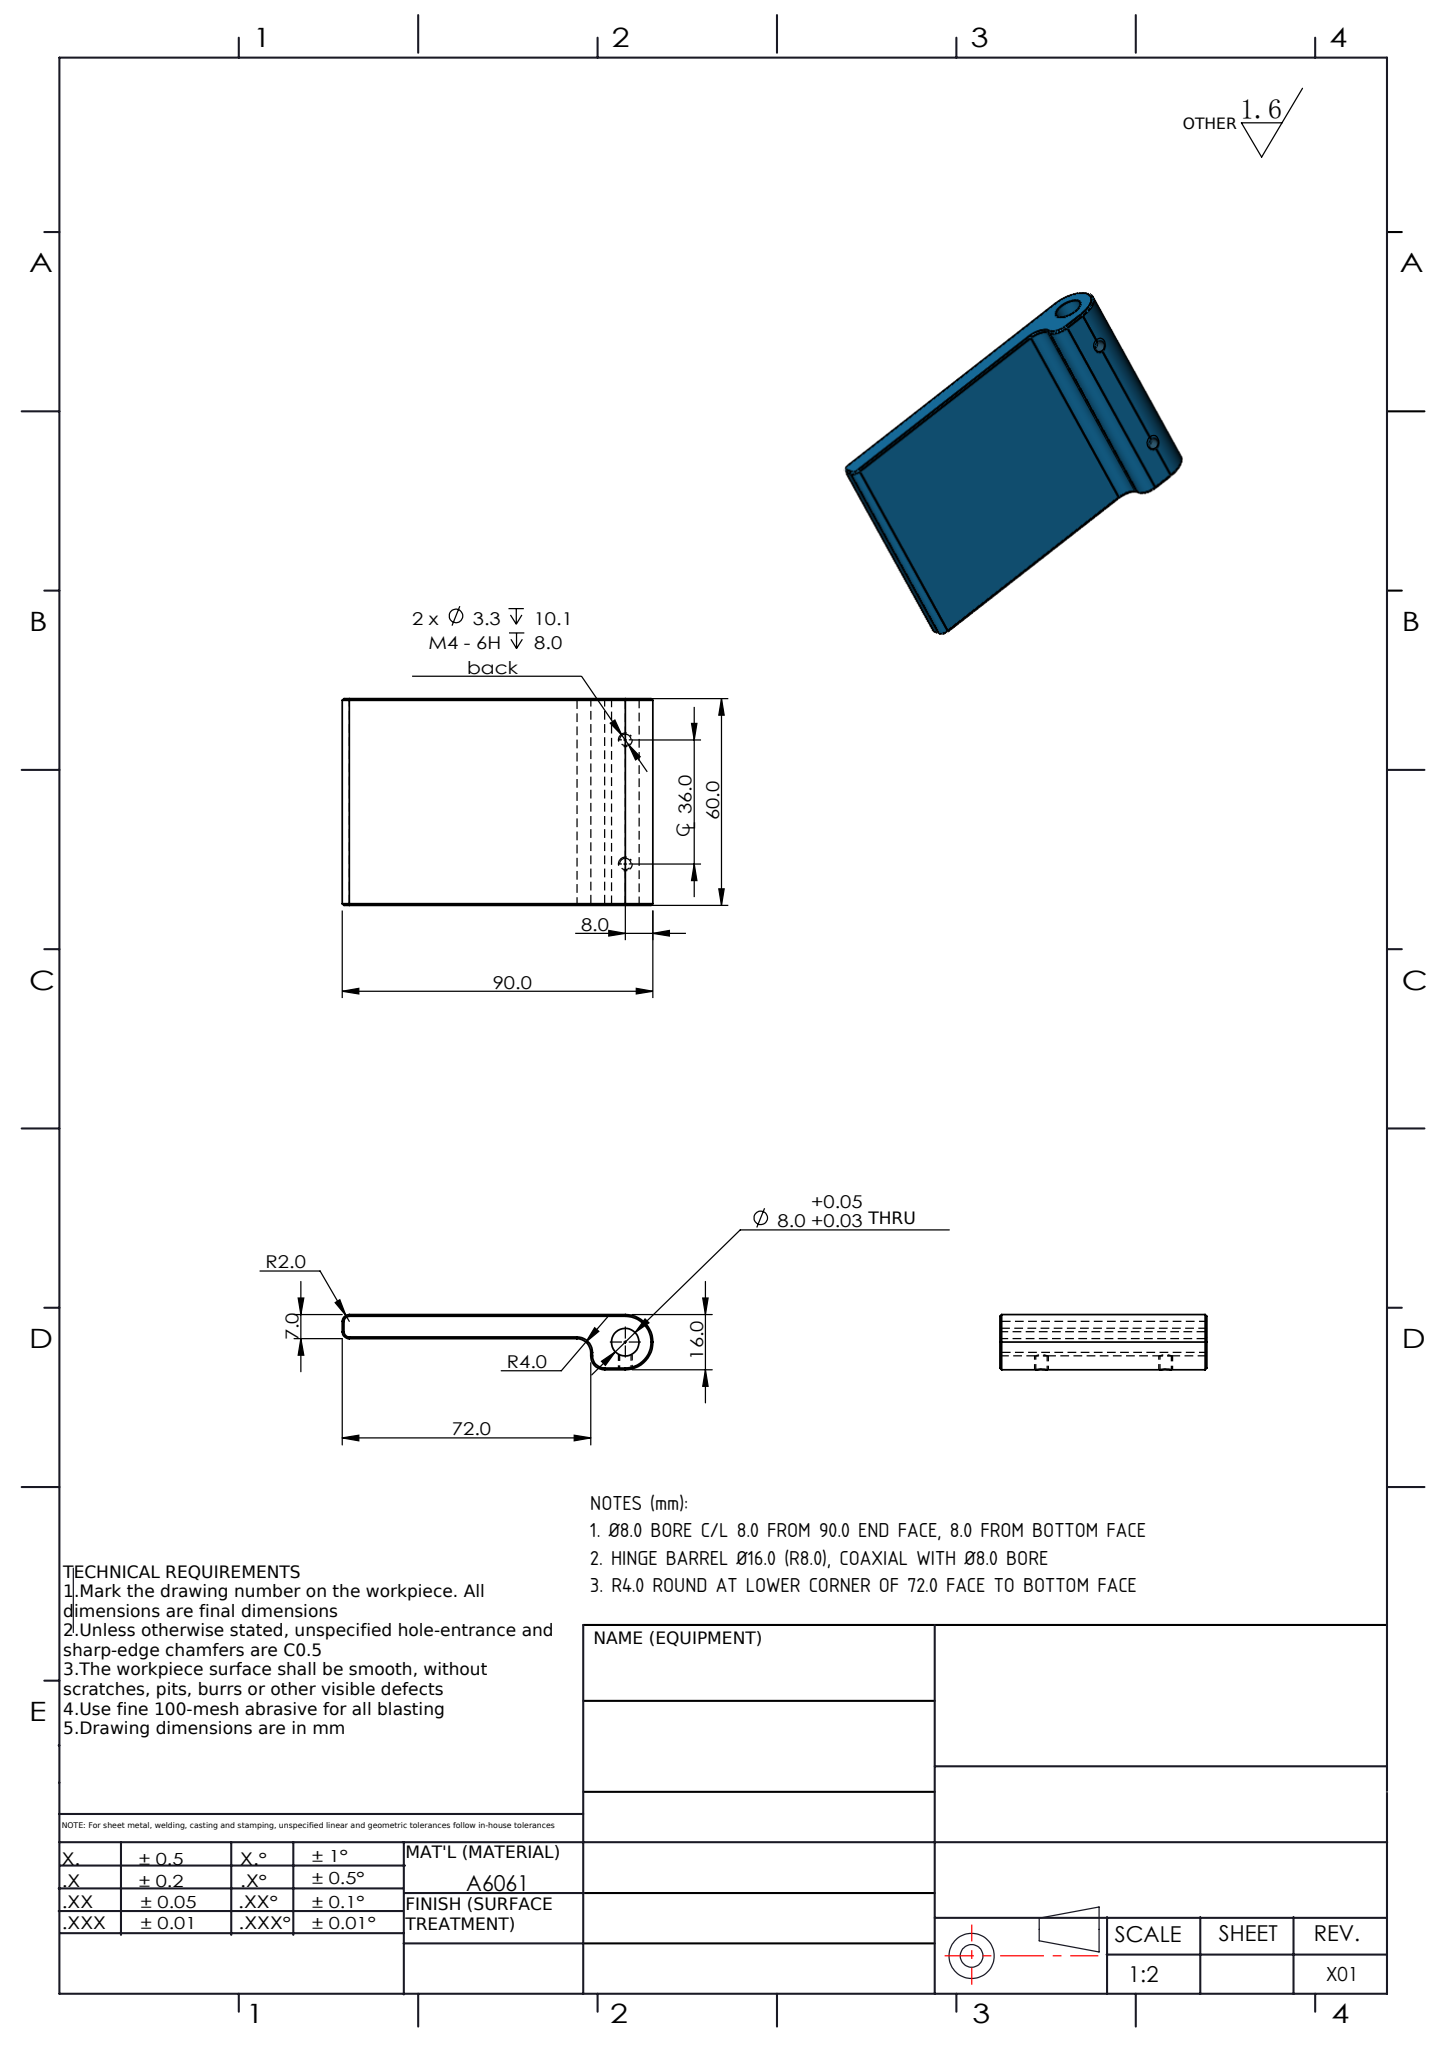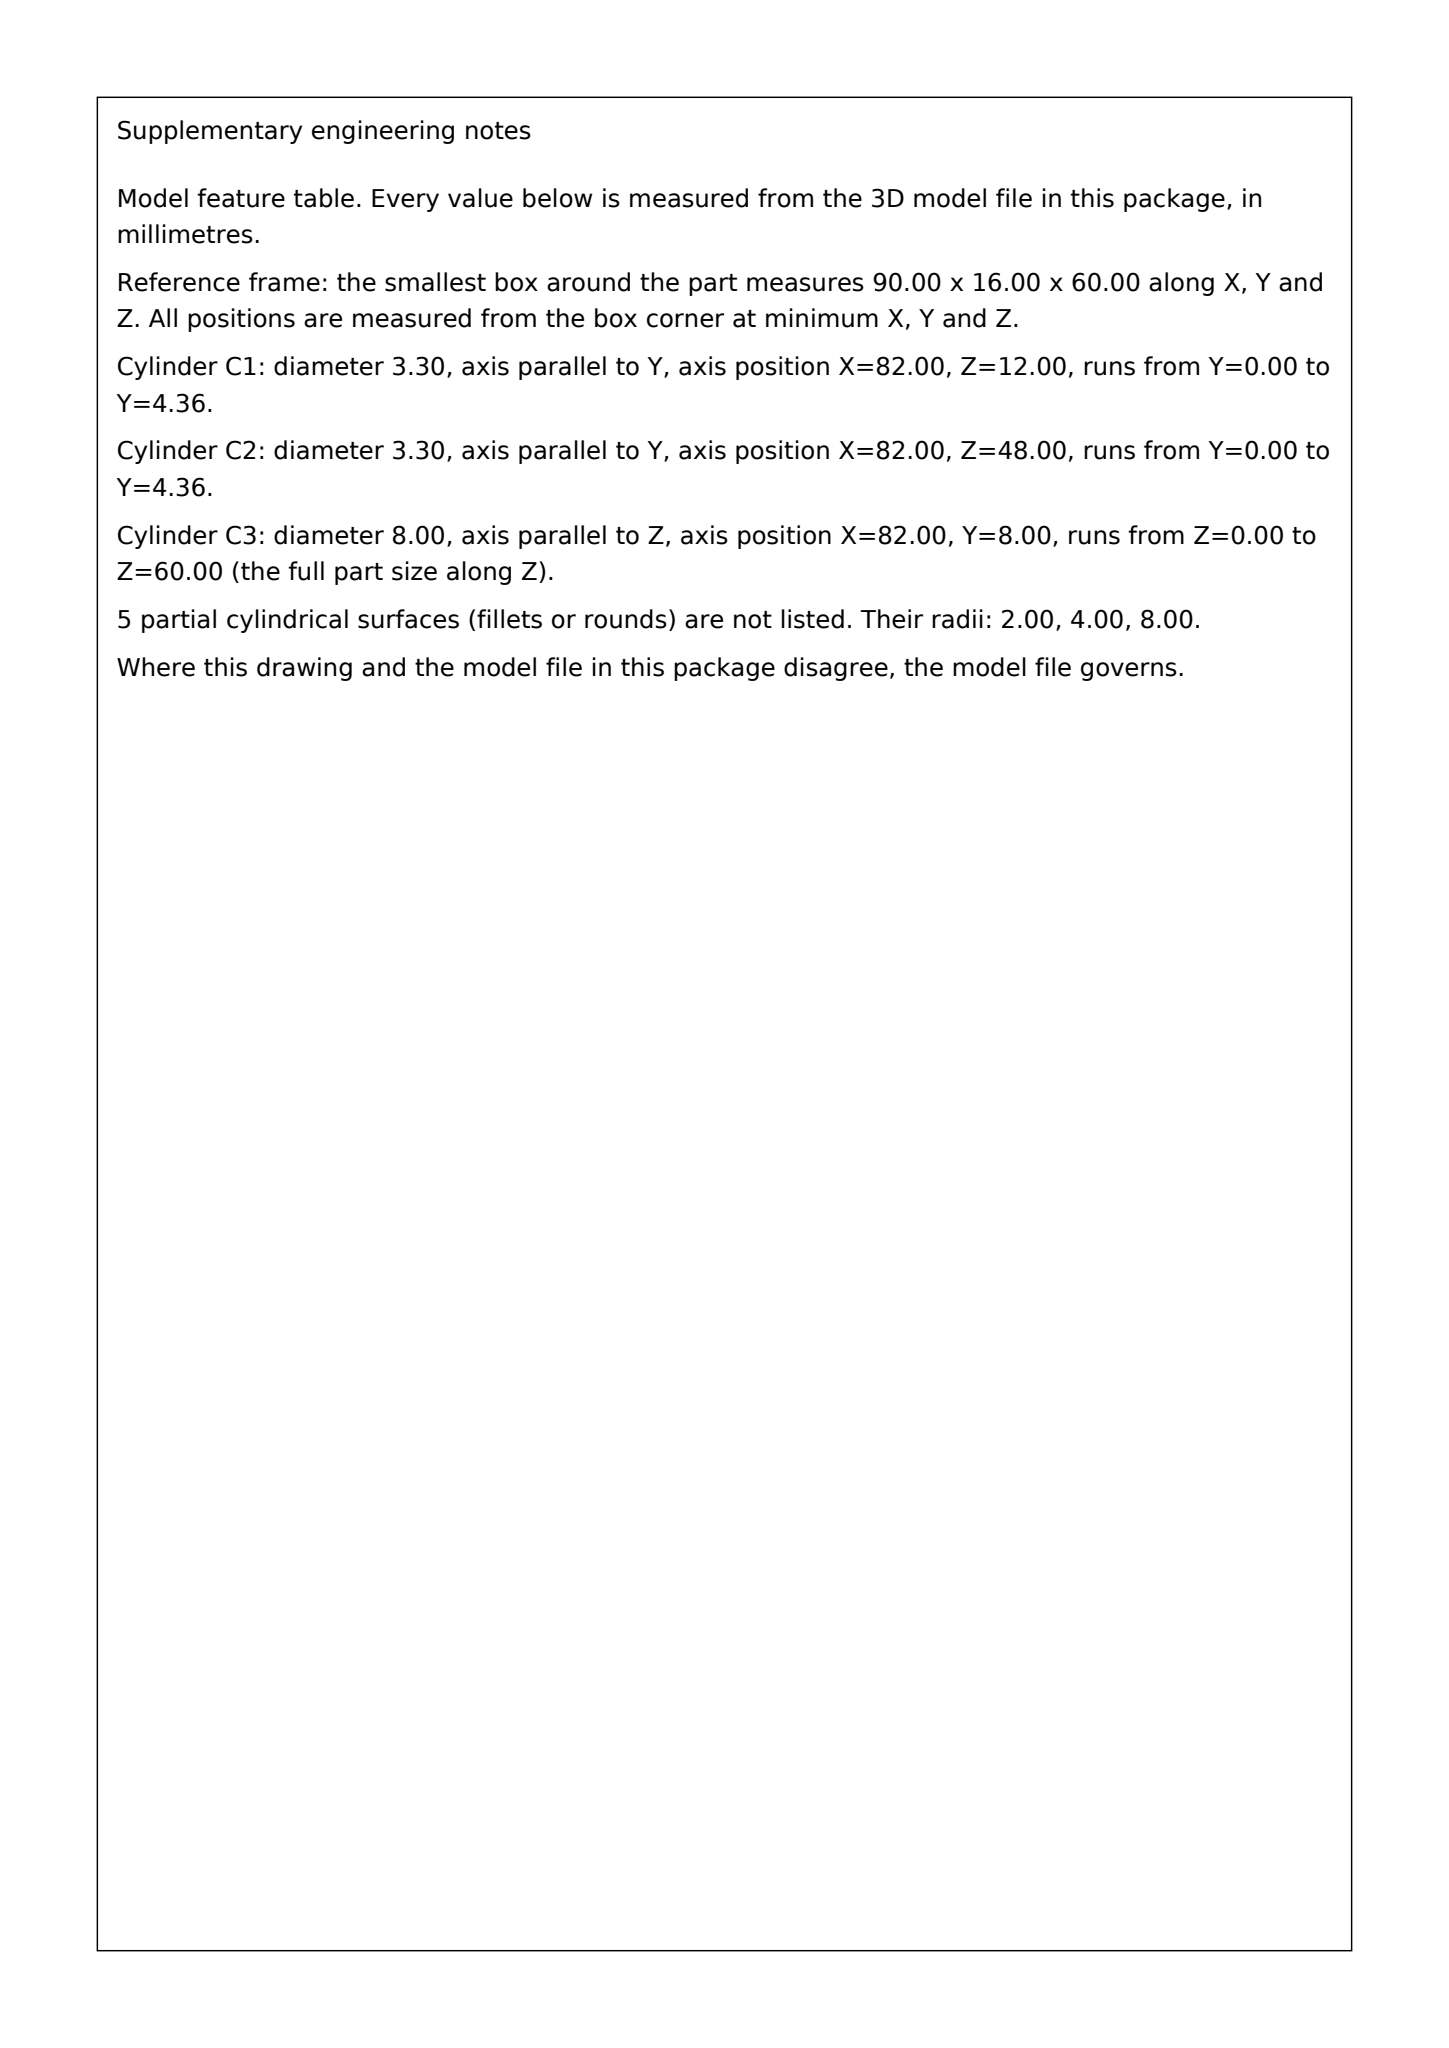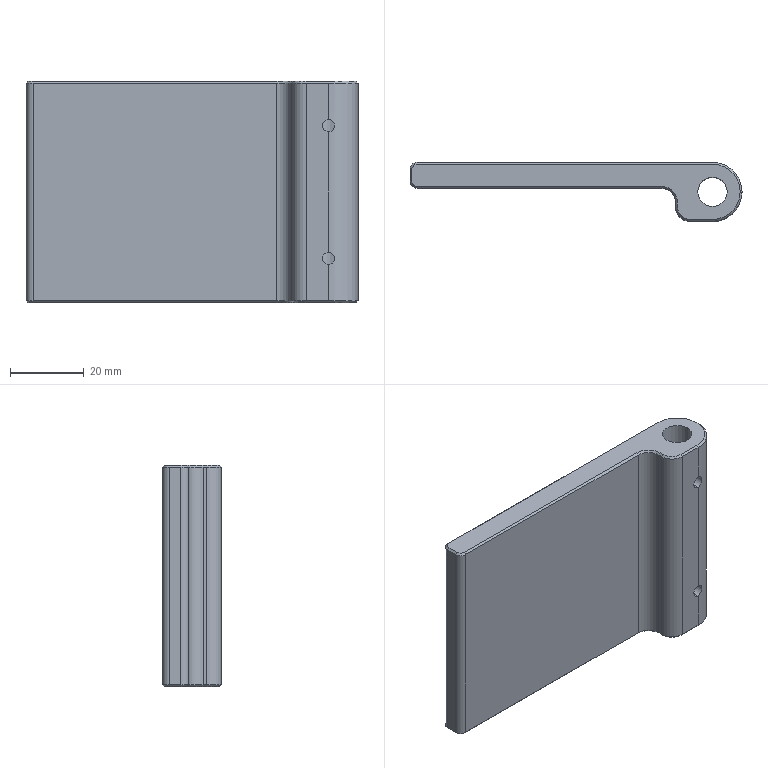Part | SolidWorks | mm | 1 solid | 41 faces | box 90 x 16 x 60 mm | volume 42634 mm3 | plane 17 | cylinder 12 | cone 12 | commonest cylinder face diameters 3.3 x4 8 x4 16 x2 4 x2
Drawing notes:
Ø8.0 BORE C/L 8.0 FROM 90.0 END FACE, 8.0 FROM BOTTOM FACE | from the solid: Ø8 THRU cyl axis z at x=82, y=8; bbox 90.0 x 16.0 -> 90-82=8 from end, 8 from bottom
HINGE BARREL Ø16.0 (R8.0), COAXIAL WITH Ø8.0 BORE | from the solid: Ø16 cyl axis z at (82,8), same axis as Ø8 THRU bore
R4.0 ROUND AT LOWER CORNER OF 72.0 FACE TO BOTTOM FACE | from the solid: Ø8 (R4) cyl axis z centred (76,4), tangent to x=72 plane and y=0 bottom face